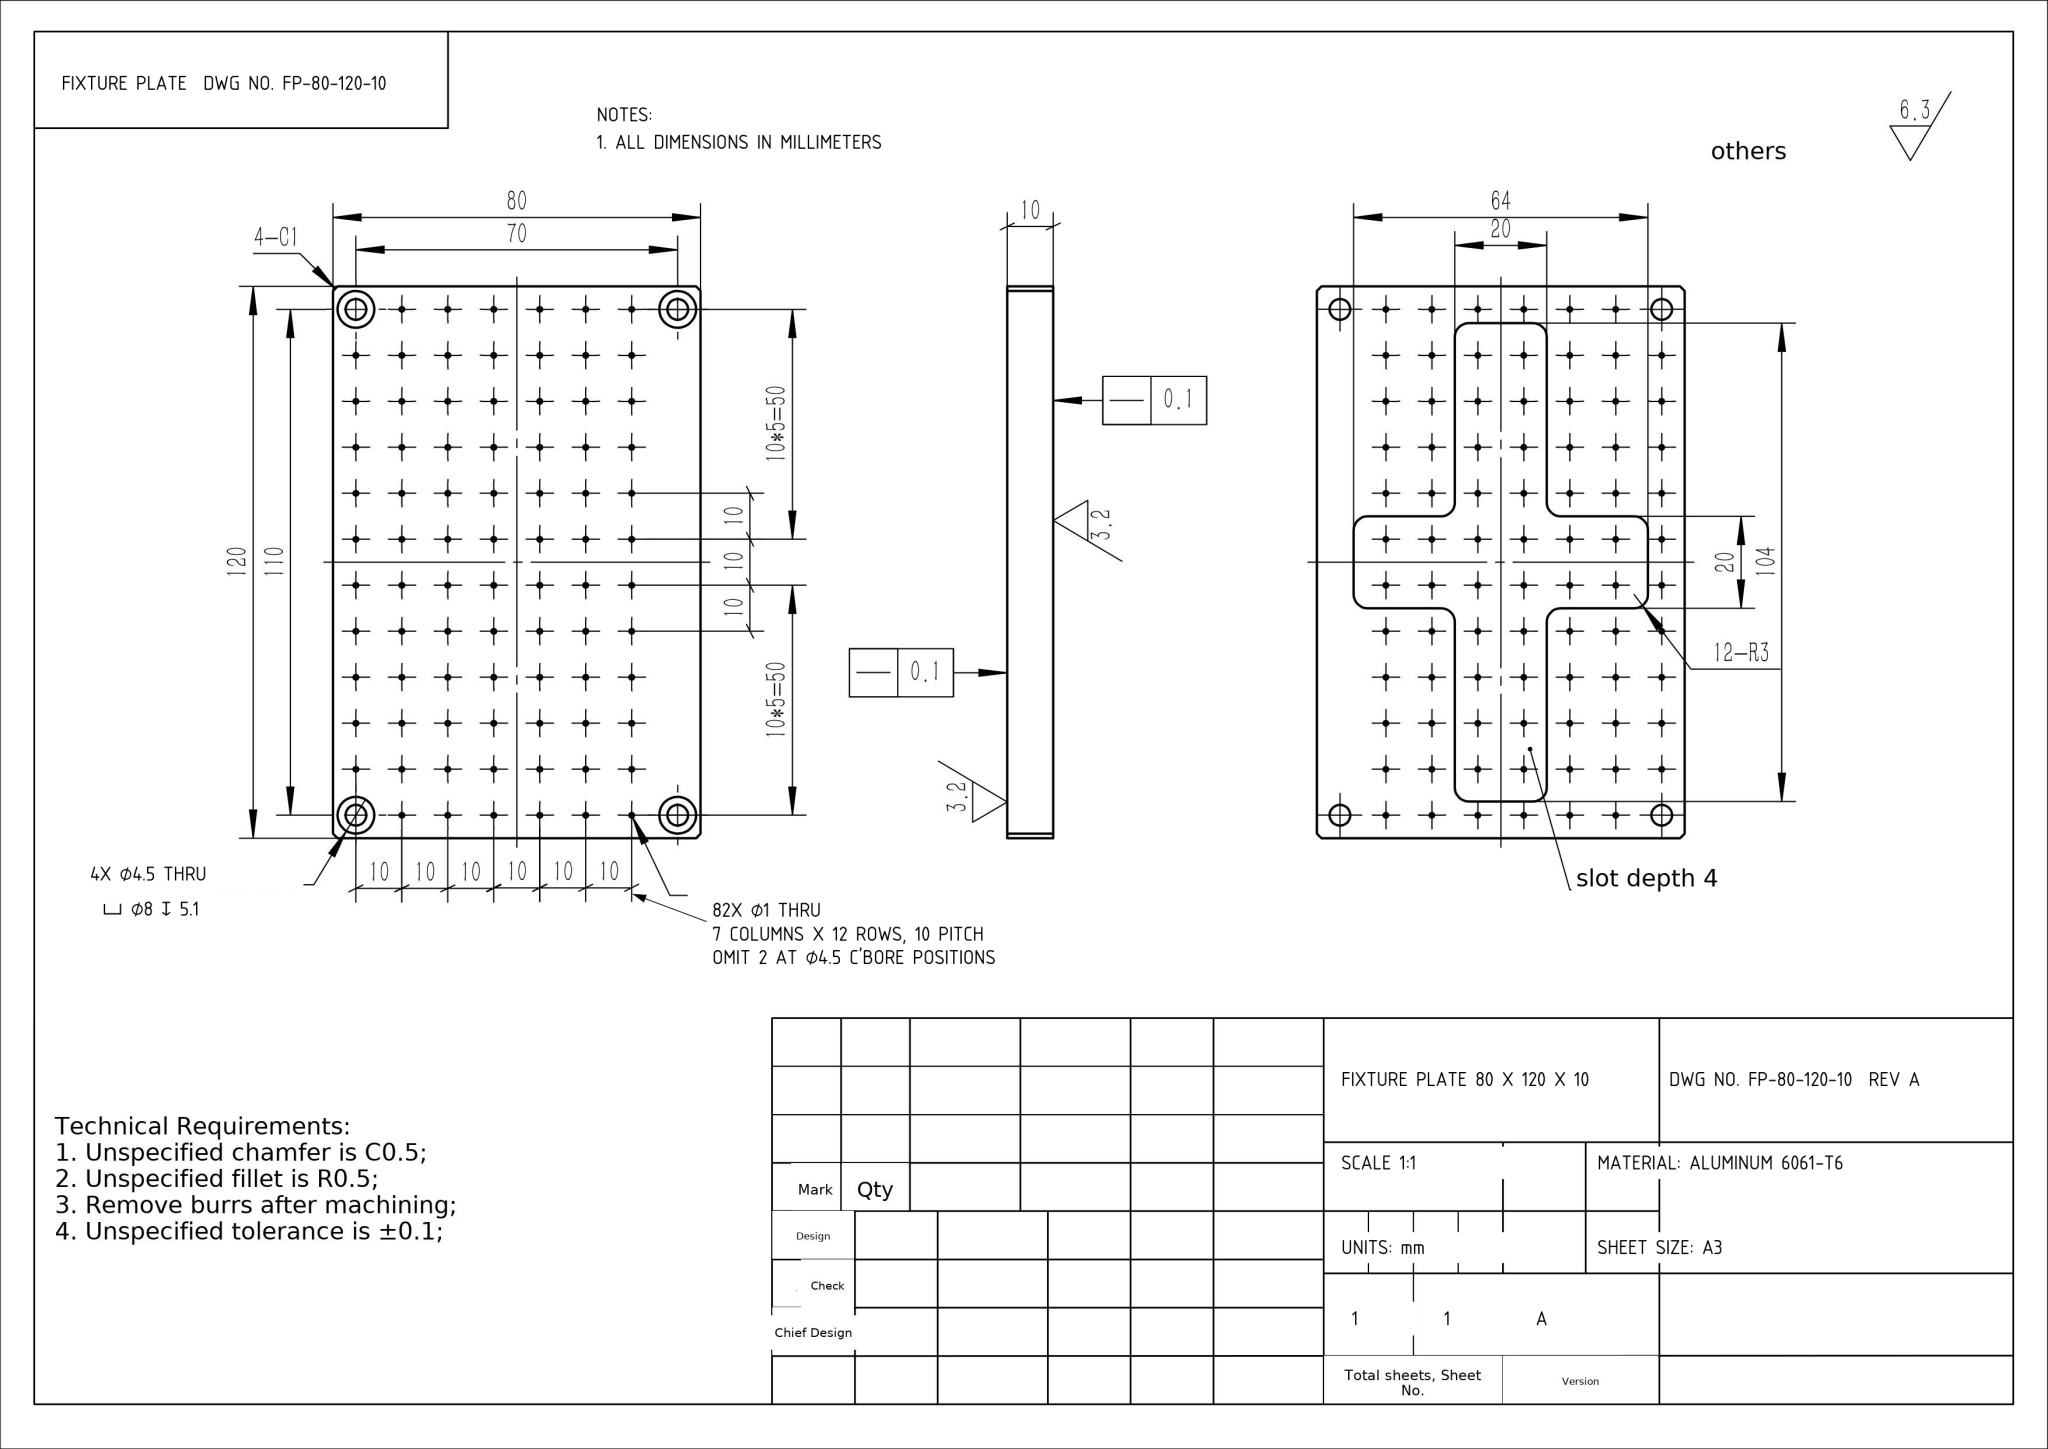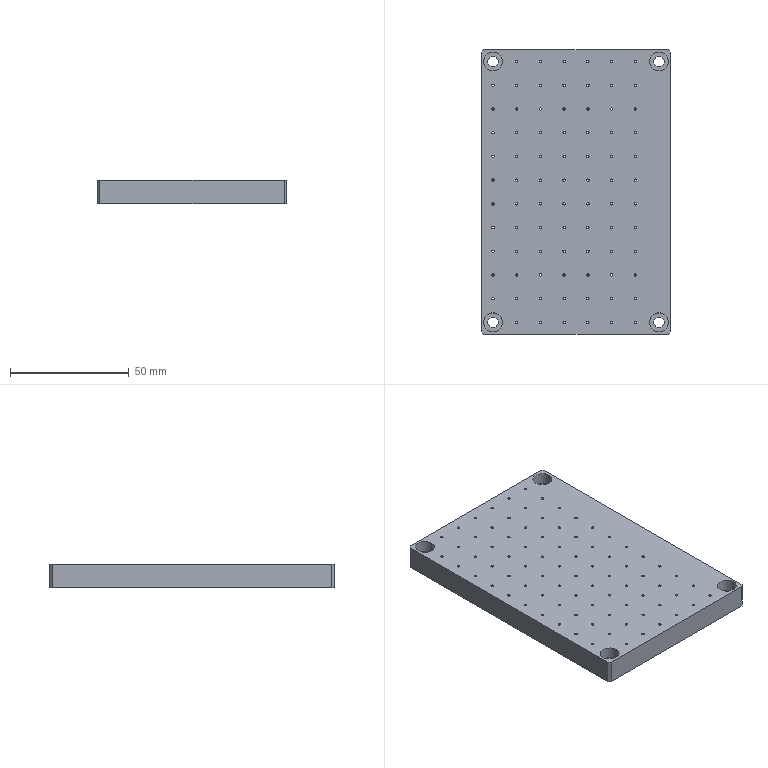Part | NX | mm | 1 solid | 219 faces | box 80 x 120 x 10 mm | volume 82278 mm3 | cylinder 192 | plane 27 | commonest cylinder face diameters 1 x164 6 x12 8 x8 4.5 x8